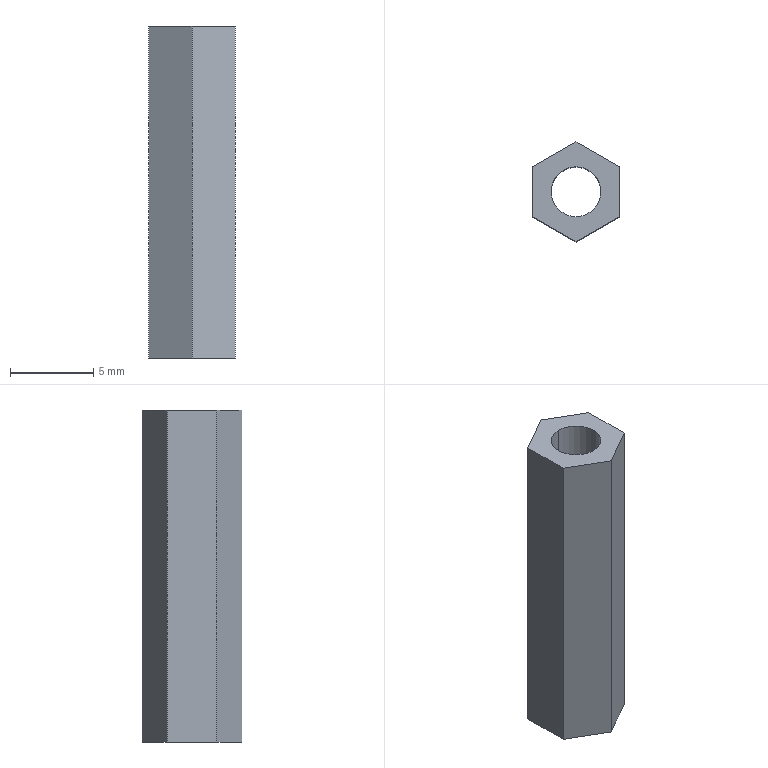Component | SolidWorks | Gimbal-1_20Pillars-1 | 1 solid | 10 faces | box 5.2 x 6 x 20 mm | volume 326 mm3 | plane 8 | cylinder 2 | commonest cylinder face diameters 3 x2
build123d program:
from build123d import *

# Parameters (mm, degrees)
SKETCH1_R           = 1.5
BOSS_EXTRUDE1_DEPTH = 20


with BuildPart() as part:
    # Sketch1 → Boss-Extrude1 (new body)
    with BuildSketch(Plane.XY):
        Polygon((3, 0), (1.5, 2.598), (-1.5, 2.598), (-3, 0), (-1.5, -2.598), (1.5, -2.598), align=None)
        Circle(SKETCH1_R, mode=Mode.SUBTRACT)
    extrude(amount=BOSS_EXTRUDE1_DEPTH)


solid = part.part

# Placed as in the assembly
solid = solid.moved(Location((26.5, 70, -20), (0, 0, 90)))
STEP:
#1=CARTESIAN_POINT('',(1.043,2.815,-0.7874));
#2=VERTEX_POINT('',#1);
#3=CARTESIAN_POINT('',(1.043,2.697,-0.7874));
#4=VERTEX_POINT('',#3);
#5=CARTESIAN_POINT('',(1.043,2.756,-0.7874));
#6=DIRECTION('',(0.,0.,-1.));
#7=DIRECTION('',(0.,-1.,0.));
#8=AXIS2_PLACEMENT_3D('',#5,#6,#7);
#9=CIRCLE('',#8,0.05906);
#10=EDGE_CURVE('',#2,#4,#9,.T.);
#11=ORIENTED_EDGE('',*,*,#10,.T.);
#12=CARTESIAN_POINT('',(1.043,2.697,0.));
#13=VERTEX_POINT('',#12);
#14=CARTESIAN_POINT('',(1.043,2.697,-0.7874));
#15=DIRECTION('',(0.,0.,1.));
#16=VECTOR('',#15,39.37);
#17=LINE('',#14,#16);
#18=EDGE_CURVE('',#4,#13,#17,.T.);
#19=ORIENTED_EDGE('',*,*,#18,.T.);
#20=CARTESIAN_POINT('',(1.043,2.815,0.));
#21=VERTEX_POINT('',#20);
#22=CARTESIAN_POINT('',(1.043,2.756,0.));
#23=DIRECTION('',(0.,0.,-1.));
#24=DIRECTION('',(0.,-1.,0.));
#25=AXIS2_PLACEMENT_3D('',#22,#23,#24);
#26=CIRCLE('',#25,0.05906);
#27=EDGE_CURVE('',#21,#13,#26,.T.);
#28=ORIENTED_EDGE('',*,*,#27,.F.);
#29=CARTESIAN_POINT('',(1.043,2.815,-0.7874));
#30=DIRECTION('',(0.,0.,1.));
#31=VECTOR('',#30,39.37);
#32=LINE('',#29,#31);
#33=EDGE_CURVE('',#2,#21,#32,.T.);
#34=ORIENTED_EDGE('',*,*,#33,.F.);
#35=EDGE_LOOP('',(#11,#19,#28,#34));
#36=FACE_OUTER_BOUND('',#35,.T.);
#37=CARTESIAN_POINT('',(1.043,2.756,-0.7874));
#38=DIRECTION('',(0.,0.,1.));
#39=DIRECTION('',(-0.,1.,0.));
#40=AXIS2_PLACEMENT_3D('',#37,#38,#39);
#41=CYLINDRICAL_SURFACE('',#40,0.05906);
#42=ADVANCED_FACE('',(#36),#41,.F.);
#43=CARTESIAN_POINT('',(1.146,2.697,-0.7874));
#44=VERTEX_POINT('',#43);
#45=CARTESIAN_POINT('',(1.043,2.638,-0.7874));
#46=VERTEX_POINT('',#45);
#47=CARTESIAN_POINT('',(1.146,2.697,-0.7874));
#48=DIRECTION('',(-0.866,-0.5,0.));
#49=VECTOR('',#48,39.37);
#50=LINE('',#47,#49);
#51=EDGE_CURVE('',#44,#46,#50,.T.);
#52=ORIENTED_EDGE('',*,*,#51,.T.);
#53=CARTESIAN_POINT('',(0.941,2.697,-0.7874));
#54=VERTEX_POINT('',#53);
#55=CARTESIAN_POINT('',(1.043,2.638,-0.7874));
#56=DIRECTION('',(-0.866,0.5,0.));
#57=VECTOR('',#56,39.37);
#58=LINE('',#55,#57);
#59=EDGE_CURVE('',#46,#54,#58,.T.);
#60=ORIENTED_EDGE('',*,*,#59,.T.);
#61=CARTESIAN_POINT('',(0.941,2.815,-0.7874));
#62=VERTEX_POINT('',#61);
#63=CARTESIAN_POINT('',(0.941,2.697,-0.7874));
#64=DIRECTION('',(-0.,1.,0.));
#65=VECTOR('',#64,39.37);
#66=LINE('',#63,#65);
#67=EDGE_CURVE('',#54,#62,#66,.T.);
#68=ORIENTED_EDGE('',*,*,#67,.T.);
#69=CARTESIAN_POINT('',(1.043,2.874,-0.7874));
#70=VERTEX_POINT('',#69);
#71=CARTESIAN_POINT('',(0.941,2.815,-0.7874));
#72=DIRECTION('',(0.866,0.5,0.));
#73=VECTOR('',#72,39.37);
#74=LINE('',#71,#73);
#75=EDGE_CURVE('',#62,#70,#74,.T.);
#76=ORIENTED_EDGE('',*,*,#75,.T.);
#77=CARTESIAN_POINT('',(1.146,2.815,-0.7874));
#78=VERTEX_POINT('',#77);
#79=CARTESIAN_POINT('',(1.043,2.874,-0.7874));
#80=DIRECTION('',(0.866,-0.5,0.));
#81=VECTOR('',#80,39.37);
#82=LINE('',#79,#81);
#83=EDGE_CURVE('',#70,#78,#82,.T.);
#84=ORIENTED_EDGE('',*,*,#83,.T.);
#85=CARTESIAN_POINT('',(1.146,2.815,-0.7874));
#86=DIRECTION('',(0.,-1.,0.));
#87=VECTOR('',#86,39.37);
#88=LINE('',#85,#87);
#89=EDGE_CURVE('',#78,#44,#88,.T.);
#90=ORIENTED_EDGE('',*,*,#89,.T.);
#91=EDGE_LOOP('',(#52,#60,#68,#76,#84,#90));
#92=FACE_OUTER_BOUND('',#91,.T.);
#93=ORIENTED_EDGE('',*,*,#10,.F.);
#94=CARTESIAN_POINT('',(1.043,2.756,-0.7874));
#95=DIRECTION('',(0.,0.,-1.));
#96=DIRECTION('',(0.,-1.,0.));
#97=AXIS2_PLACEMENT_3D('',#94,#95,#96);
#98=CIRCLE('',#97,0.05906);
#99=EDGE_CURVE('',#4,#2,#98,.T.);
#100=ORIENTED_EDGE('',*,*,#99,.F.);
#101=EDGE_LOOP('',(#93,#100));
#102=FACE_BOUND('',#101,.T.);
#103=CARTESIAN_POINT('',(1.043,2.756,-0.7874));
#104=DIRECTION('',(0.,0.,-1.));
#105=DIRECTION('',(0.,-1.,0.));
#106=AXIS2_PLACEMENT_3D('',#103,#104,#105);
#107=PLANE('',#106);
#108=ADVANCED_FACE('',(#92,#102),#107,.T.);
#109=CARTESIAN_POINT('',(1.146,2.697,0.));
#110=VERTEX_POINT('',#109);
#111=CARTESIAN_POINT('',(1.043,2.638,0.));
#112=VERTEX_POINT('',#111);
#113=CARTESIAN_POINT('',(1.146,2.697,0.));
#114=DIRECTION('',(-0.866,-0.5,0.));
#115=VECTOR('',#114,39.37);
#116=LINE('',#113,#115);
#117=EDGE_CURVE('',#110,#112,#116,.T.);
#118=ORIENTED_EDGE('',*,*,#117,.F.);
#119=CARTESIAN_POINT('',(1.146,2.815,0.));
#120=VERTEX_POINT('',#119);
#121=CARTESIAN_POINT('',(1.146,2.815,0.));
#122=DIRECTION('',(0.,-1.,0.));
#123=VECTOR('',#122,39.37);
#124=LINE('',#121,#123);
#125=EDGE_CURVE('',#120,#110,#124,.T.);
#126=ORIENTED_EDGE('',*,*,#125,.F.);
#127=CARTESIAN_POINT('',(1.043,2.874,0.));
#128=VERTEX_POINT('',#127);
#129=CARTESIAN_POINT('',(1.043,2.874,0.));
#130=DIRECTION('',(0.866,-0.5,0.));
#131=VECTOR('',#130,39.37);
#132=LINE('',#129,#131);
#133=EDGE_CURVE('',#128,#120,#132,.T.);
#134=ORIENTED_EDGE('',*,*,#133,.F.);
#135=CARTESIAN_POINT('',(0.941,2.815,0.));
#136=VERTEX_POINT('',#135);
#137=CARTESIAN_POINT('',(0.941,2.815,0.));
#138=DIRECTION('',(0.866,0.5,0.));
#139=VECTOR('',#138,39.37);
#140=LINE('',#137,#139);
#141=EDGE_CURVE('',#136,#128,#140,.T.);
#142=ORIENTED_EDGE('',*,*,#141,.F.);
#143=CARTESIAN_POINT('',(0.941,2.697,0.));
#144=VERTEX_POINT('',#143);
#145=CARTESIAN_POINT('',(0.941,2.697,0.));
#146=DIRECTION('',(-0.,1.,0.));
#147=VECTOR('',#146,39.37);
#148=LINE('',#145,#147);
#149=EDGE_CURVE('',#144,#136,#148,.T.);
#150=ORIENTED_EDGE('',*,*,#149,.F.);
#151=CARTESIAN_POINT('',(1.043,2.638,0.));
#152=DIRECTION('',(-0.866,0.5,0.));
#153=VECTOR('',#152,39.37);
#154=LINE('',#151,#153);
#155=EDGE_CURVE('',#112,#144,#154,.T.);
#156=ORIENTED_EDGE('',*,*,#155,.F.);
#157=EDGE_LOOP('',(#118,#126,#134,#142,#150,#156));
#158=FACE_OUTER_BOUND('',#157,.T.);
#159=ORIENTED_EDGE('',*,*,#27,.T.);
#160=CARTESIAN_POINT('',(1.043,2.756,0.));
#161=DIRECTION('',(0.,0.,-1.));
#162=DIRECTION('',(0.,-1.,0.));
#163=AXIS2_PLACEMENT_3D('',#160,#161,#162);
#164=CIRCLE('',#163,0.05906);
#165=EDGE_CURVE('',#13,#21,#164,.T.);
#166=ORIENTED_EDGE('',*,*,#165,.T.);
#167=EDGE_LOOP('',(#159,#166));
#168=FACE_BOUND('',#167,.T.);
#169=CARTESIAN_POINT('',(1.043,2.756,0.));
#170=DIRECTION('',(0.,0.,-1.));
#171=DIRECTION('',(0.,-1.,0.));
#172=AXIS2_PLACEMENT_3D('',#169,#170,#171);
#173=PLANE('',#172);
#174=ADVANCED_FACE('',(#158,#168),#173,.F.);
#175=ORIENTED_EDGE('',*,*,#117,.T.);
#176=CARTESIAN_POINT('',(1.043,2.638,-0.7874));
#177=DIRECTION('',(0.,0.,1.));
#178=VECTOR('',#177,39.37);
#179=LINE('',#176,#178);
#180=EDGE_CURVE('',#46,#112,#179,.T.);
#181=ORIENTED_EDGE('',*,*,#180,.F.);
#182=ORIENTED_EDGE('',*,*,#51,.F.);
#183=CARTESIAN_POINT('',(1.146,2.697,-0.7874));
#184=DIRECTION('',(0.,0.,1.));
#185=VECTOR('',#184,39.37);
#186=LINE('',#183,#185);
#187=EDGE_CURVE('',#44,#110,#186,.T.);
#188=ORIENTED_EDGE('',*,*,#187,.T.);
#189=EDGE_LOOP('',(#175,#181,#182,#188));
#190=FACE_OUTER_BOUND('',#189,.T.);
#191=CARTESIAN_POINT('',(1.146,2.697,-0.7874));
#192=DIRECTION('',(-0.5,0.866,0.));
#193=DIRECTION('',(0.866,0.5,0.));
#194=AXIS2_PLACEMENT_3D('',#191,#192,#193);
#195=PLANE('',#194);
#196=ADVANCED_FACE('',(#190),#195,.F.);
#197=ORIENTED_EDGE('',*,*,#155,.T.);
#198=CARTESIAN_POINT('',(0.941,2.697,-0.7874));
#199=DIRECTION('',(0.,0.,1.));
#200=VECTOR('',#199,39.37);
#201=LINE('',#198,#200);
#202=EDGE_CURVE('',#54,#144,#201,.T.);
#203=ORIENTED_EDGE('',*,*,#202,.F.);
#204=ORIENTED_EDGE('',*,*,#59,.F.);
#205=ORIENTED_EDGE('',*,*,#180,.T.);
#206=EDGE_LOOP('',(#197,#203,#204,#205));
#207=FACE_OUTER_BOUND('',#206,.T.);
#208=CARTESIAN_POINT('',(1.043,2.638,-0.7874));
#209=DIRECTION('',(0.5,0.866,0.));
#210=DIRECTION('',(0.866,-0.5,0.));
#211=AXIS2_PLACEMENT_3D('',#208,#209,#210);
#212=PLANE('',#211);
#213=ADVANCED_FACE('',(#207),#212,.F.);
#214=ORIENTED_EDGE('',*,*,#149,.T.);
#215=CARTESIAN_POINT('',(0.941,2.815,-0.7874));
#216=DIRECTION('',(0.,0.,1.));
#217=VECTOR('',#216,39.37);
#218=LINE('',#215,#217);
#219=EDGE_CURVE('',#62,#136,#218,.T.);
#220=ORIENTED_EDGE('',*,*,#219,.F.);
#221=ORIENTED_EDGE('',*,*,#67,.F.);
#222=ORIENTED_EDGE('',*,*,#202,.T.);
#223=EDGE_LOOP('',(#214,#220,#221,#222));
#224=FACE_OUTER_BOUND('',#223,.T.);
#225=CARTESIAN_POINT('',(0.941,2.697,-0.7874));
#226=DIRECTION('',(1.,0.,0.));
#227=DIRECTION('',(0.,-1.,0.));
#228=AXIS2_PLACEMENT_3D('',#225,#226,#227);
#229=PLANE('',#228);
#230=ADVANCED_FACE('',(#224),#229,.F.);
#231=ORIENTED_EDGE('',*,*,#141,.T.);
#232=CARTESIAN_POINT('',(1.043,2.874,-0.7874));
#233=DIRECTION('',(0.,0.,1.));
#234=VECTOR('',#233,39.37);
#235=LINE('',#232,#234);
#236=EDGE_CURVE('',#70,#128,#235,.T.);
#237=ORIENTED_EDGE('',*,*,#236,.F.);
#238=ORIENTED_EDGE('',*,*,#75,.F.);
#239=ORIENTED_EDGE('',*,*,#219,.T.);
#240=EDGE_LOOP('',(#231,#237,#238,#239));
#241=FACE_OUTER_BOUND('',#240,.T.);
#242=CARTESIAN_POINT('',(0.941,2.815,-0.7874));
#243=DIRECTION('',(0.5,-0.866,0.));
#244=DIRECTION('',(-0.866,-0.5,0.));
#245=AXIS2_PLACEMENT_3D('',#242,#243,#244);
#246=PLANE('',#245);
#247=ADVANCED_FACE('',(#241),#246,.F.);
#248=ORIENTED_EDGE('',*,*,#133,.T.);
#249=CARTESIAN_POINT('',(1.146,2.815,-0.7874));
#250=DIRECTION('',(0.,0.,1.));
#251=VECTOR('',#250,39.37);
#252=LINE('',#249,#251);
#253=EDGE_CURVE('',#78,#120,#252,.T.);
#254=ORIENTED_EDGE('',*,*,#253,.F.);
#255=ORIENTED_EDGE('',*,*,#83,.F.);
#256=ORIENTED_EDGE('',*,*,#236,.T.);
#257=EDGE_LOOP('',(#248,#254,#255,#256));
#258=FACE_OUTER_BOUND('',#257,.T.);
#259=CARTESIAN_POINT('',(1.043,2.874,-0.7874));
#260=DIRECTION('',(-0.5,-0.866,0.));
#261=DIRECTION('',(-0.866,0.5,0.));
#262=AXIS2_PLACEMENT_3D('',#259,#260,#261);
#263=PLANE('',#262);
#264=ADVANCED_FACE('',(#258),#263,.F.);
#265=ORIENTED_EDGE('',*,*,#125,.T.);
#266=ORIENTED_EDGE('',*,*,#187,.F.);
#267=ORIENTED_EDGE('',*,*,#89,.F.);
#268=ORIENTED_EDGE('',*,*,#253,.T.);
#269=EDGE_LOOP('',(#265,#266,#267,#268));
#270=FACE_OUTER_BOUND('',#269,.T.);
#271=CARTESIAN_POINT('',(1.146,2.815,-0.7874));
#272=DIRECTION('',(-1.,-0.,0.));
#273=DIRECTION('',(-0.,1.,0.));
#274=AXIS2_PLACEMENT_3D('',#271,#272,#273);
#275=PLANE('',#274);
#276=ADVANCED_FACE('',(#270),#275,.F.);
#277=ORIENTED_EDGE('',*,*,#18,.F.);
#278=ORIENTED_EDGE('',*,*,#99,.T.);
#279=ORIENTED_EDGE('',*,*,#33,.T.);
#280=ORIENTED_EDGE('',*,*,#165,.F.);
#281=EDGE_LOOP('',(#277,#278,#279,#280));
#282=FACE_OUTER_BOUND('',#281,.T.);
#283=CARTESIAN_POINT('',(1.043,2.756,-0.7874));
#284=DIRECTION('',(0.,0.,1.));
#285=DIRECTION('',(-0.,1.,0.));
#286=AXIS2_PLACEMENT_3D('',#283,#284,#285);
#287=CYLINDRICAL_SURFACE('',#286,0.05906);
#288=ADVANCED_FACE('',(#282),#287,.F.);
#289=CLOSED_SHELL('',(#42,#108,#174,#196,#213,#230,#247,#264,#276,#288));
#290=MANIFOLD_SOLID_BREP('',#289);
#291=CARTESIAN_POINT('',(0.,0.,0.));
#292=DIRECTION('',(0.,0.,1.));
#293=DIRECTION('',(1.,0.,0.));
#294=AXIS2_PLACEMENT_3D('',#291,#292,#293);
#295=(LENGTH_UNIT()NAMED_UNIT(*)SI_UNIT($,.METRE.));
#296=LENGTH_MEASURE_WITH_UNIT(LENGTH_MEASURE(0.0254),#295);
#297=DIMENSIONAL_EXPONENTS(1.,0.,0.,0.,0.,0.,0.);
#298=(CONVERSION_BASED_UNIT('',#296)LENGTH_UNIT()NAMED_UNIT(#297));
#299=UNCERTAINTY_MEASURE_WITH_UNIT(LENGTH_MEASURE(0.00001),#298,'','');
#300=(NAMED_UNIT(*)PLANE_ANGLE_UNIT()SI_UNIT($,.RADIAN.));
#301=(NAMED_UNIT(*)SI_UNIT($,.STERADIAN.)SOLID_ANGLE_UNIT());
#302=(GEOMETRIC_REPRESENTATION_CONTEXT(3)GLOBAL_UNCERTAINTY_ASSIGNED_CONTEXT((#299))GLOBAL_UNIT_ASSIGNED_CONTEXT((#298,#300,#301))REPRESENTATION_CONTEXT('',''));
#303=ADVANCED_BREP_SHAPE_REPRESENTATION('',(#290,#294),#302);
#304=COLOUR_RGB('',0.7922,0.8196,0.9333);
#305=FILL_AREA_STYLE_COLOUR('',#304);
#306=FILL_AREA_STYLE('',(#305));
#307=SURFACE_STYLE_FILL_AREA(#306);
#308=SURFACE_SIDE_STYLE('',(#307));
#309=SURFACE_STYLE_USAGE(.BOTH.,#308);
#310=PRESENTATION_STYLE_ASSIGNMENT((#309));
#311=STYLED_ITEM('',(#310),#290);
#312=(LENGTH_UNIT()NAMED_UNIT(*)SI_UNIT($,.METRE.));
#313=LENGTH_MEASURE_WITH_UNIT(LENGTH_MEASURE(0.0254),#312);
#314=DIMENSIONAL_EXPONENTS(1.,0.,0.,0.,0.,0.,0.);
#315=(CONVERSION_BASED_UNIT('',#313)LENGTH_UNIT()NAMED_UNIT(#314));
#316=UNCERTAINTY_MEASURE_WITH_UNIT(LENGTH_MEASURE(0.00001),#315,'','');
#317=(NAMED_UNIT(*)PLANE_ANGLE_UNIT()SI_UNIT($,.RADIAN.));
#318=(NAMED_UNIT(*)SI_UNIT($,.STERADIAN.)SOLID_ANGLE_UNIT());
#319=(GEOMETRIC_REPRESENTATION_CONTEXT(3)GLOBAL_UNCERTAINTY_ASSIGNED_CONTEXT((#316))GLOBAL_UNIT_ASSIGNED_CONTEXT((#315,#317,#318))REPRESENTATION_CONTEXT('',''));
#320=MECHANICAL_DESIGN_GEOMETRIC_PRESENTATION_REPRESENTATION('',(#311),#319);
#321=PRESENTATION_LAYER_ASSIGNMENT('','',(#311));